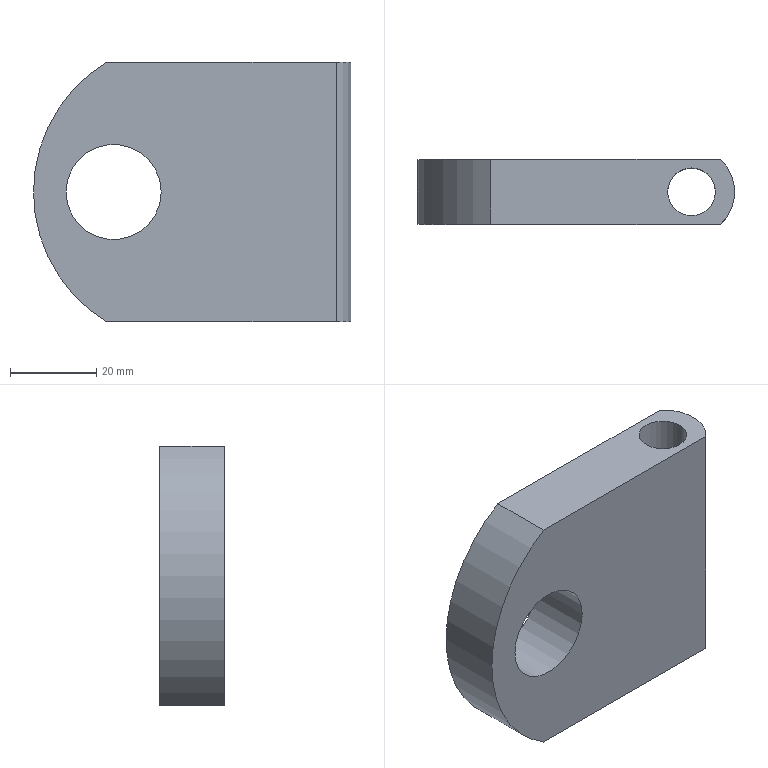Component | NX | MODEL2 | 1 solid | 8 faces | box 73.39 x 15 x 60 mm | volume 49250 mm3 | plane 4 | cylinder 4 | commonest cylinder face diameters 20 x1 11 x1 70.098 x1 22 x1
STEP:
#1=CARTESIAN_POINT('',(0.,0.,0.));
#2=DIRECTION('',(0.,0.,1.));
#3=DIRECTION('',(1.,0.,0.));
#4=AXIS2_PLACEMENT_3D('',#1,#2,#3);
#5=CARTESIAN_POINT('',(-84.997,-51.411,30.));
#6=VERTEX_POINT('',#5);
#7=CARTESIAN_POINT('',(-84.997,-56.911,30.));
#8=DIRECTION('',(0.,0.,1.));
#9=DIRECTION('',(0.,1.,0.));
#10=AXIS2_PLACEMENT_3D('',#7,#8,#9);
#11=CIRCLE('',#10,5.5);
#12=CARTESIAN_POINT('',(-84.997,-56.911,30.));
#13=DIRECTION('',(0.,0.,1.));
#14=DIRECTION('',(1.,0.,0.));
#15=AXIS2_PLACEMENT_3D('',#12,#13,#14);
#16=PLANE('',#15);
#17=CARTESIAN_POINT('',(0.,0.));
#18=DIRECTION('',(0.,1.));
#19=AXIS2_PLACEMENT_2D('',#17,#18);
#20=CIRCLE('',#19,5.5);
#21=(GEOMETRIC_REPRESENTATION_CONTEXT(2)PARAMETRIC_REPRESENTATION_CONTEXT()REPRESENTATION_CONTEXT('',''));
#22=DEFINITIONAL_REPRESENTATION('',(#20),#21);
#23=PCURVE('',#16,#22);
#24=CARTESIAN_POINT('',(-84.997,-56.911,30.));
#25=DIRECTION('',(0.,0.,-1.));
#26=DIRECTION('',(-1.,0.,0.));
#27=AXIS2_PLACEMENT_3D('',#24,#25,#26);
#28=CYLINDRICAL_SURFACE('',#27,5.5);
#29=CARTESIAN_POINT('',(7.854,0.));
#30=DIRECTION('',(-1.,0.));
#31=VECTOR('',#30,1.);
#32=LINE('',#29,#31);
#33=(GEOMETRIC_REPRESENTATION_CONTEXT(2)PARAMETRIC_REPRESENTATION_CONTEXT()REPRESENTATION_CONTEXT('',''));
#34=DEFINITIONAL_REPRESENTATION('',(#32),#33);
#35=PCURVE('',#28,#34);
#36=SURFACE_CURVE('',#11,(#23,#35),.PCURVE_S1.);
#37=EDGE_CURVE('',#6,#6,#36,.T.);
#38=ORIENTED_EDGE('',*,*,#37,.F.);
#39=EDGE_LOOP('',(#38));
#40=FACE_BOUND('',#39,.T.);
#41=CARTESIAN_POINT('',(-78.382,-49.411,30.));
#42=VERTEX_POINT('',#41);
#43=CARTESIAN_POINT('',(-131.456,-49.411,30.));
#44=VERTEX_POINT('',#43);
#45=CARTESIAN_POINT('',(-78.382,-49.411,30.));
#46=DIRECTION('',(-1.,0.,0.));
#47=VECTOR('',#46,1.);
#48=LINE('',#45,#47);
#49=CARTESIAN_POINT('',(6.614,7.5));
#50=DIRECTION('',(-1.,0.));
#51=VECTOR('',#50,1.);
#52=LINE('',#49,#51);
#53=(GEOMETRIC_REPRESENTATION_CONTEXT(2)PARAMETRIC_REPRESENTATION_CONTEXT()REPRESENTATION_CONTEXT('',''));
#54=DEFINITIONAL_REPRESENTATION('',(#52),#53);
#55=PCURVE('',#16,#54);
#56=CARTESIAN_POINT('',(-78.382,-49.411,30.));
#57=DIRECTION('',(-0.,-1.,0.));
#58=DIRECTION('',(1.,-0.,0.));
#59=AXIS2_PLACEMENT_3D('',#56,#57,#58);
#60=PLANE('',#59);
#61=CARTESIAN_POINT('',(0.,0.));
#62=DIRECTION('',(-1.,0.));
#63=VECTOR('',#62,1.);
#64=LINE('',#61,#63);
#65=(GEOMETRIC_REPRESENTATION_CONTEXT(2)PARAMETRIC_REPRESENTATION_CONTEXT()REPRESENTATION_CONTEXT('',''));
#66=DEFINITIONAL_REPRESENTATION('',(#64),#65);
#67=PCURVE('',#60,#66);
#68=SURFACE_CURVE('',#48,(#55,#67),.PCURVE_S1.);
#69=EDGE_CURVE('',#42,#44,#68,.T.);
#70=ORIENTED_EDGE('',*,*,#69,.T.);
#71=CARTESIAN_POINT('',(-131.456,-64.411,30.));
#72=VERTEX_POINT('',#71);
#73=CARTESIAN_POINT('',(-131.456,-19.411,30.));
#74=DIRECTION('',(0.,-1.,0.));
#75=VECTOR('',#74,1.);
#76=LINE('',#73,#75);
#77=CARTESIAN_POINT('',(-46.459,37.5));
#78=DIRECTION('',(0.,-1.));
#79=VECTOR('',#78,1.);
#80=LINE('',#77,#79);
#81=(GEOMETRIC_REPRESENTATION_CONTEXT(2)PARAMETRIC_REPRESENTATION_CONTEXT()REPRESENTATION_CONTEXT('',''));
#82=DEFINITIONAL_REPRESENTATION('',(#80),#81);
#83=PCURVE('',#16,#82);
#84=CARTESIAN_POINT('',(-113.333,-19.411,-0.));
#85=DIRECTION('',(0.,-1.,0.));
#86=DIRECTION('',(1.,0.,0.));
#87=AXIS2_PLACEMENT_3D('',#84,#85,#86);
#88=CYLINDRICAL_SURFACE('',#87,35.049);
#89=CARTESIAN_POINT('',(2.114,0.));
#90=DIRECTION('',(0.,1.));
#91=VECTOR('',#90,1.);
#92=LINE('',#89,#91);
#93=(GEOMETRIC_REPRESENTATION_CONTEXT(2)PARAMETRIC_REPRESENTATION_CONTEXT()REPRESENTATION_CONTEXT('',''));
#94=DEFINITIONAL_REPRESENTATION('',(#92),#93);
#95=PCURVE('',#88,#94);
#96=SURFACE_CURVE('',#76,(#83,#95),.PCURVE_S1.);
#97=EDGE_CURVE('',#44,#72,#96,.T.);
#98=ORIENTED_EDGE('',*,*,#97,.T.);
#99=CARTESIAN_POINT('',(-78.382,-64.411,30.));
#100=VERTEX_POINT('',#99);
#101=CARTESIAN_POINT('',(-148.382,-64.411,30.));
#102=DIRECTION('',(1.,0.,0.));
#103=VECTOR('',#102,1.);
#104=LINE('',#101,#103);
#105=CARTESIAN_POINT('',(-63.386,-7.5));
#106=DIRECTION('',(1.,0.));
#107=VECTOR('',#106,1.);
#108=LINE('',#105,#107);
#109=(GEOMETRIC_REPRESENTATION_CONTEXT(2)PARAMETRIC_REPRESENTATION_CONTEXT()REPRESENTATION_CONTEXT('',''));
#110=DEFINITIONAL_REPRESENTATION('',(#108),#109);
#111=PCURVE('',#16,#110);
#112=CARTESIAN_POINT('',(-148.382,-64.411,30.));
#113=DIRECTION('',(-0.,1.,0.));
#114=DIRECTION('',(-1.,-0.,0.));
#115=AXIS2_PLACEMENT_3D('',#112,#113,#114);
#116=PLANE('',#115);
#117=CARTESIAN_POINT('',(0.,0.));
#118=DIRECTION('',(-1.,0.));
#119=VECTOR('',#118,1.);
#120=LINE('',#117,#119);
#121=(GEOMETRIC_REPRESENTATION_CONTEXT(2)PARAMETRIC_REPRESENTATION_CONTEXT()REPRESENTATION_CONTEXT('',''));
#122=DEFINITIONAL_REPRESENTATION('',(#120),#121);
#123=PCURVE('',#116,#122);
#124=SURFACE_CURVE('',#104,(#111,#123),.PCURVE_S1.);
#125=EDGE_CURVE('',#72,#100,#124,.T.);
#126=ORIENTED_EDGE('',*,*,#125,.T.);
#127=CARTESIAN_POINT('',(-84.997,-56.911,30.));
#128=DIRECTION('',(0.,0.,1.));
#129=DIRECTION('',(0.,1.,0.));
#130=AXIS2_PLACEMENT_3D('',#127,#128,#129);
#131=CIRCLE('',#130,10.);
#132=CARTESIAN_POINT('',(0.,0.));
#133=DIRECTION('',(0.,1.));
#134=AXIS2_PLACEMENT_2D('',#132,#133);
#135=CIRCLE('',#134,10.);
#136=(GEOMETRIC_REPRESENTATION_CONTEXT(2)PARAMETRIC_REPRESENTATION_CONTEXT()REPRESENTATION_CONTEXT('',''));
#137=DEFINITIONAL_REPRESENTATION('',(#135),#136);
#138=PCURVE('',#16,#137);
#139=CARTESIAN_POINT('',(-84.997,-56.911,30.));
#140=DIRECTION('',(0.,0.,-1.));
#141=DIRECTION('',(-1.,0.,0.));
#142=AXIS2_PLACEMENT_3D('',#139,#140,#141);
#143=CYLINDRICAL_SURFACE('',#142,10.);
#144=CARTESIAN_POINT('',(7.854,0.));
#145=DIRECTION('',(-1.,0.));
#146=VECTOR('',#145,1.);
#147=LINE('',#144,#146);
#148=(GEOMETRIC_REPRESENTATION_CONTEXT(2)PARAMETRIC_REPRESENTATION_CONTEXT()REPRESENTATION_CONTEXT('',''));
#149=DEFINITIONAL_REPRESENTATION('',(#147),#148);
#150=PCURVE('',#143,#149);
#151=SURFACE_CURVE('',#131,(#138,#150),.PCURVE_S1.);
#152=EDGE_CURVE('',#100,#42,#151,.T.);
#153=ORIENTED_EDGE('',*,*,#152,.T.);
#154=EDGE_LOOP('',(#70,#98,#126,#153));
#155=FACE_BOUND('',#154,.T.);
#156=ADVANCED_FACE('',(#40,#155),#16,.T.);
#157=CARTESIAN_POINT('',(-84.997,-51.411,-30.));
#158=VERTEX_POINT('',#157);
#159=CARTESIAN_POINT('',(-84.997,-56.911,-30.));
#160=DIRECTION('',(0.,0.,1.));
#161=DIRECTION('',(0.,1.,0.));
#162=AXIS2_PLACEMENT_3D('',#159,#160,#161);
#163=CIRCLE('',#162,5.5);
#164=CARTESIAN_POINT('',(-84.997,-56.911,-30.));
#165=DIRECTION('',(0.,0.,1.));
#166=DIRECTION('',(1.,0.,0.));
#167=AXIS2_PLACEMENT_3D('',#164,#165,#166);
#168=PLANE('',#167);
#169=CARTESIAN_POINT('',(0.,0.));
#170=DIRECTION('',(0.,1.));
#171=AXIS2_PLACEMENT_2D('',#169,#170);
#172=CIRCLE('',#171,5.5);
#173=(GEOMETRIC_REPRESENTATION_CONTEXT(2)PARAMETRIC_REPRESENTATION_CONTEXT()REPRESENTATION_CONTEXT('',''));
#174=DEFINITIONAL_REPRESENTATION('',(#172),#173);
#175=PCURVE('',#168,#174);
#176=CARTESIAN_POINT('',(7.854,60.));
#177=DIRECTION('',(-1.,0.));
#178=VECTOR('',#177,1.);
#179=LINE('',#176,#178);
#180=(GEOMETRIC_REPRESENTATION_CONTEXT(2)PARAMETRIC_REPRESENTATION_CONTEXT()REPRESENTATION_CONTEXT('',''));
#181=DEFINITIONAL_REPRESENTATION('',(#179),#180);
#182=PCURVE('',#28,#181);
#183=SURFACE_CURVE('',#163,(#175,#182),.PCURVE_S1.);
#184=EDGE_CURVE('',#158,#158,#183,.T.);
#185=ORIENTED_EDGE('',*,*,#184,.T.);
#186=EDGE_LOOP('',(#185));
#187=FACE_BOUND('',#186,.T.);
#188=CARTESIAN_POINT('',(-131.456,-49.411,-30.));
#189=VERTEX_POINT('',#188);
#190=CARTESIAN_POINT('',(-131.456,-64.411,-30.));
#191=VERTEX_POINT('',#190);
#192=CARTESIAN_POINT('',(-131.456,-19.411,-30.));
#193=DIRECTION('',(0.,-1.,0.));
#194=VECTOR('',#193,1.);
#195=LINE('',#192,#194);
#196=CARTESIAN_POINT('',(-46.459,37.5));
#197=DIRECTION('',(0.,-1.));
#198=VECTOR('',#197,1.);
#199=LINE('',#196,#198);
#200=(GEOMETRIC_REPRESENTATION_CONTEXT(2)PARAMETRIC_REPRESENTATION_CONTEXT()REPRESENTATION_CONTEXT('',''));
#201=DEFINITIONAL_REPRESENTATION('',(#199),#200);
#202=PCURVE('',#168,#201);
#203=CARTESIAN_POINT('',(4.169,0.));
#204=DIRECTION('',(0.,1.));
#205=VECTOR('',#204,1.);
#206=LINE('',#203,#205);
#207=(GEOMETRIC_REPRESENTATION_CONTEXT(2)PARAMETRIC_REPRESENTATION_CONTEXT()REPRESENTATION_CONTEXT('',''));
#208=DEFINITIONAL_REPRESENTATION('',(#206),#207);
#209=PCURVE('',#88,#208);
#210=SURFACE_CURVE('',#195,(#202,#209),.PCURVE_S1.);
#211=EDGE_CURVE('',#189,#191,#210,.T.);
#212=ORIENTED_EDGE('',*,*,#211,.F.);
#213=CARTESIAN_POINT('',(-78.382,-49.411,-30.));
#214=VERTEX_POINT('',#213);
#215=CARTESIAN_POINT('',(-78.382,-49.411,-30.));
#216=DIRECTION('',(-1.,0.,0.));
#217=VECTOR('',#216,1.);
#218=LINE('',#215,#217);
#219=CARTESIAN_POINT('',(6.614,7.5));
#220=DIRECTION('',(-1.,0.));
#221=VECTOR('',#220,1.);
#222=LINE('',#219,#221);
#223=(GEOMETRIC_REPRESENTATION_CONTEXT(2)PARAMETRIC_REPRESENTATION_CONTEXT()REPRESENTATION_CONTEXT('',''));
#224=DEFINITIONAL_REPRESENTATION('',(#222),#223);
#225=PCURVE('',#168,#224);
#226=CARTESIAN_POINT('',(0.,-60.));
#227=DIRECTION('',(-1.,0.));
#228=VECTOR('',#227,1.);
#229=LINE('',#226,#228);
#230=(GEOMETRIC_REPRESENTATION_CONTEXT(2)PARAMETRIC_REPRESENTATION_CONTEXT()REPRESENTATION_CONTEXT('',''));
#231=DEFINITIONAL_REPRESENTATION('',(#229),#230);
#232=PCURVE('',#60,#231);
#233=SURFACE_CURVE('',#218,(#225,#232),.PCURVE_S1.);
#234=EDGE_CURVE('',#214,#189,#233,.T.);
#235=ORIENTED_EDGE('',*,*,#234,.F.);
#236=CARTESIAN_POINT('',(-78.382,-64.411,-30.));
#237=VERTEX_POINT('',#236);
#238=CARTESIAN_POINT('',(-84.997,-56.911,-30.));
#239=DIRECTION('',(0.,0.,1.));
#240=DIRECTION('',(0.,1.,0.));
#241=AXIS2_PLACEMENT_3D('',#238,#239,#240);
#242=CIRCLE('',#241,10.);
#243=CARTESIAN_POINT('',(0.,0.));
#244=DIRECTION('',(0.,1.));
#245=AXIS2_PLACEMENT_2D('',#243,#244);
#246=CIRCLE('',#245,10.);
#247=(GEOMETRIC_REPRESENTATION_CONTEXT(2)PARAMETRIC_REPRESENTATION_CONTEXT()REPRESENTATION_CONTEXT('',''));
#248=DEFINITIONAL_REPRESENTATION('',(#246),#247);
#249=PCURVE('',#168,#248);
#250=CARTESIAN_POINT('',(7.854,60.));
#251=DIRECTION('',(-1.,0.));
#252=VECTOR('',#251,1.);
#253=LINE('',#250,#252);
#254=(GEOMETRIC_REPRESENTATION_CONTEXT(2)PARAMETRIC_REPRESENTATION_CONTEXT()REPRESENTATION_CONTEXT('',''));
#255=DEFINITIONAL_REPRESENTATION('',(#253),#254);
#256=PCURVE('',#143,#255);
#257=SURFACE_CURVE('',#242,(#249,#256),.PCURVE_S1.);
#258=EDGE_CURVE('',#237,#214,#257,.T.);
#259=ORIENTED_EDGE('',*,*,#258,.F.);
#260=CARTESIAN_POINT('',(-148.382,-64.411,-30.));
#261=DIRECTION('',(1.,0.,0.));
#262=VECTOR('',#261,1.);
#263=LINE('',#260,#262);
#264=CARTESIAN_POINT('',(-63.386,-7.5));
#265=DIRECTION('',(1.,0.));
#266=VECTOR('',#265,1.);
#267=LINE('',#264,#266);
#268=(GEOMETRIC_REPRESENTATION_CONTEXT(2)PARAMETRIC_REPRESENTATION_CONTEXT()REPRESENTATION_CONTEXT('',''));
#269=DEFINITIONAL_REPRESENTATION('',(#267),#268);
#270=PCURVE('',#168,#269);
#271=CARTESIAN_POINT('',(0.,-60.));
#272=DIRECTION('',(-1.,0.));
#273=VECTOR('',#272,1.);
#274=LINE('',#271,#273);
#275=(GEOMETRIC_REPRESENTATION_CONTEXT(2)PARAMETRIC_REPRESENTATION_CONTEXT()REPRESENTATION_CONTEXT('',''));
#276=DEFINITIONAL_REPRESENTATION('',(#274),#275);
#277=PCURVE('',#116,#276);
#278=SURFACE_CURVE('',#263,(#270,#277),.PCURVE_S1.);
#279=EDGE_CURVE('',#191,#237,#278,.T.);
#280=ORIENTED_EDGE('',*,*,#279,.F.);
#281=EDGE_LOOP('',(#212,#235,#259,#280));
#282=FACE_BOUND('',#281,.T.);
#283=ADVANCED_FACE('',(#187,#282),#168,.F.);
#284=CARTESIAN_POINT('',(-118.847,-49.411,-0.));
#285=VERTEX_POINT('',#284);
#286=CARTESIAN_POINT('',(-129.847,-49.411,-0.));
#287=DIRECTION('',(0.,1.,0.));
#288=DIRECTION('',(1.,-0.,0.));
#289=AXIS2_PLACEMENT_3D('',#286,#287,#288);
#290=CIRCLE('',#289,11.);
#291=CARTESIAN_POINT('',(-40.464,-30.));
#292=CARTESIAN_POINT('',(-40.464,-49.053));
#293=CARTESIAN_POINT('',(-56.964,-39.526));
#294=CARTESIAN_POINT('',(-73.464,-30.));
#295=CARTESIAN_POINT('',(-56.964,-20.474));
#296=CARTESIAN_POINT('',(-40.464,-10.947));
#297=CARTESIAN_POINT('',(-40.464,-30.));
#298=(BOUNDED_CURVE()B_SPLINE_CURVE(2,(#291,#292,#293,#294,#295,#296,#297),.UNSPECIFIED.,.T.,.F.)B_SPLINE_CURVE_WITH_KNOTS((1,2,2,2,2,1),(-2.094,0.,2.094,4.189,6.283,8.378),.UNSPECIFIED.)CURVE()GEOMETRIC_REPRESENTATION_ITEM()RATIONAL_B_SPLINE_CURVE((1.,0.5,1.,0.5,1.,0.5,1.))REPRESENTATION_ITEM(''));
#299=(GEOMETRIC_REPRESENTATION_CONTEXT(2)PARAMETRIC_REPRESENTATION_CONTEXT()REPRESENTATION_CONTEXT('',''));
#300=DEFINITIONAL_REPRESENTATION('',(#298),#299);
#301=PCURVE('',#60,#300);
#302=CARTESIAN_POINT('',(-129.847,-19.411,-0.));
#303=DIRECTION('',(0.,-1.,0.));
#304=DIRECTION('',(1.,0.,0.));
#305=AXIS2_PLACEMENT_3D('',#302,#303,#304);
#306=CYLINDRICAL_SURFACE('',#305,11.);
#307=CARTESIAN_POINT('',(6.283,30.));
#308=DIRECTION('',(-1.,0.));
#309=VECTOR('',#308,1.);
#310=LINE('',#307,#309);
#311=(GEOMETRIC_REPRESENTATION_CONTEXT(2)PARAMETRIC_REPRESENTATION_CONTEXT()REPRESENTATION_CONTEXT('',''));
#312=DEFINITIONAL_REPRESENTATION('',(#310),#311);
#313=PCURVE('',#306,#312);
#314=SURFACE_CURVE('',#290,(#301,#313),.PCURVE_S1.);
#315=EDGE_CURVE('',#285,#285,#314,.T.);
#316=ORIENTED_EDGE('',*,*,#315,.F.);
#317=EDGE_LOOP('',(#316));
#318=FACE_BOUND('',#317,.T.);
#319=CARTESIAN_POINT('',(-113.333,-49.411,-0.));
#320=DIRECTION('',(-0.,-1.,0.));
#321=DIRECTION('',(1.,-0.,0.));
#322=AXIS2_PLACEMENT_3D('',#319,#320,#321);
#323=CIRCLE('',#322,35.049);
#324=CARTESIAN_POINT('',(-34.951,-30.));
#325=DIRECTION('',(1.,0.));
#326=AXIS2_PLACEMENT_2D('',#324,#325);
#327=CIRCLE('',#326,35.049);
#328=(GEOMETRIC_REPRESENTATION_CONTEXT(2)PARAMETRIC_REPRESENTATION_CONTEXT()REPRESENTATION_CONTEXT('',''));
#329=DEFINITIONAL_REPRESENTATION('',(#327),#328);
#330=PCURVE('',#60,#329);
#331=CARTESIAN_POINT('',(-0.,30.));
#332=DIRECTION('',(1.,0.));
#333=VECTOR('',#332,1.);
#334=LINE('',#331,#333);
#335=(GEOMETRIC_REPRESENTATION_CONTEXT(2)PARAMETRIC_REPRESENTATION_CONTEXT()REPRESENTATION_CONTEXT('',''));
#336=DEFINITIONAL_REPRESENTATION('',(#334),#335);
#337=PCURVE('',#88,#336);
#338=SURFACE_CURVE('',#323,(#330,#337),.PCURVE_S1.);
#339=EDGE_CURVE('',#44,#189,#338,.T.);
#340=ORIENTED_EDGE('',*,*,#339,.F.);
#341=ORIENTED_EDGE('',*,*,#69,.F.);
#342=CARTESIAN_POINT('',(-78.382,-49.411,30.));
#343=DIRECTION('',(0.,0.,-1.));
#344=VECTOR('',#343,1.);
#345=LINE('',#342,#344);
#346=CARTESIAN_POINT('',(0.,0.));
#347=DIRECTION('',(0.,-1.));
#348=VECTOR('',#347,1.);
#349=LINE('',#346,#348);
#350=(GEOMETRIC_REPRESENTATION_CONTEXT(2)PARAMETRIC_REPRESENTATION_CONTEXT()REPRESENTATION_CONTEXT('',''));
#351=DEFINITIONAL_REPRESENTATION('',(#349),#350);
#352=PCURVE('',#60,#351);
#353=CARTESIAN_POINT('',(2.294,0.));
#354=DIRECTION('',(0.,1.));
#355=VECTOR('',#354,1.);
#356=LINE('',#353,#355);
#357=(GEOMETRIC_REPRESENTATION_CONTEXT(2)PARAMETRIC_REPRESENTATION_CONTEXT()REPRESENTATION_CONTEXT('',''));
#358=DEFINITIONAL_REPRESENTATION('',(#356),#357);
#359=PCURVE('',#143,#358);
#360=SURFACE_CURVE('',#345,(#352,#359),.PCURVE_S1.);
#361=EDGE_CURVE('',#42,#214,#360,.T.);
#362=ORIENTED_EDGE('',*,*,#361,.T.);
#363=ORIENTED_EDGE('',*,*,#234,.T.);
#364=EDGE_LOOP('',(#340,#341,#362,#363));
#365=FACE_BOUND('',#364,.T.);
#366=ADVANCED_FACE('',(#318,#365),#60,.F.);
#367=CARTESIAN_POINT('',(-140.847,-64.411,-0.));
#368=VERTEX_POINT('',#367);
#369=CARTESIAN_POINT('',(-118.847,-64.411,-0.));
#370=VERTEX_POINT('',#369);
#371=CARTESIAN_POINT('',(-129.847,-64.411,-0.));
#372=DIRECTION('',(0.,-1.,0.));
#373=DIRECTION('',(-1.,-0.,0.));
#374=AXIS2_PLACEMENT_3D('',#371,#372,#373);
#375=CIRCLE('',#374,11.);
#376=CARTESIAN_POINT('',(-7.536,-30.));
#377=CARTESIAN_POINT('',(-7.536,-49.053));
#378=CARTESIAN_POINT('',(-24.036,-39.526));
#379=CARTESIAN_POINT('',(-40.536,-30.));
#380=CARTESIAN_POINT('',(-24.036,-20.474));
#381=CARTESIAN_POINT('',(-7.536,-10.947));
#382=CARTESIAN_POINT('',(-7.536,-30.));
#383=(BOUNDED_CURVE()B_SPLINE_CURVE(2,(#376,#377,#378,#379,#380,#381,#382),.UNSPECIFIED.,.T.,.F.)B_SPLINE_CURVE_WITH_KNOTS((1,2,2,2,2,1),(-2.094,0.,2.094,4.189,6.283,8.378),.UNSPECIFIED.)CURVE()GEOMETRIC_REPRESENTATION_ITEM()RATIONAL_B_SPLINE_CURVE((1.,0.5,1.,0.5,1.,0.5,1.))REPRESENTATION_ITEM(''));
#384=(GEOMETRIC_REPRESENTATION_CONTEXT(2)PARAMETRIC_REPRESENTATION_CONTEXT()REPRESENTATION_CONTEXT('',''));
#385=DEFINITIONAL_REPRESENTATION('',(#383),#384);
#386=PCURVE('',#116,#385);
#387=CARTESIAN_POINT('',(3.142,45.));
#388=DIRECTION('',(1.,0.));
#389=VECTOR('',#388,1.);
#390=LINE('',#387,#389);
#391=(GEOMETRIC_REPRESENTATION_CONTEXT(2)PARAMETRIC_REPRESENTATION_CONTEXT()REPRESENTATION_CONTEXT('',''));
#392=DEFINITIONAL_REPRESENTATION('',(#390),#391);
#393=PCURVE('',#306,#392);
#394=SURFACE_CURVE('',#375,(#386,#393),.PCURVE_S1.);
#395=EDGE_CURVE('',#368,#370,#394,.T.);
#396=ORIENTED_EDGE('',*,*,#395,.F.);
#397=CARTESIAN_POINT('',(-129.847,-64.411,-0.));
#398=DIRECTION('',(0.,-1.,0.));
#399=DIRECTION('',(-1.,-0.,0.));
#400=AXIS2_PLACEMENT_3D('',#397,#398,#399);
#401=CIRCLE('',#400,11.);
#402=CARTESIAN_POINT('',(-7.536,-30.));
#403=CARTESIAN_POINT('',(-7.536,-49.053));
#404=CARTESIAN_POINT('',(-24.036,-39.526));
#405=CARTESIAN_POINT('',(-40.536,-30.));
#406=CARTESIAN_POINT('',(-24.036,-20.474));
#407=CARTESIAN_POINT('',(-7.536,-10.947));
#408=CARTESIAN_POINT('',(-7.536,-30.));
#409=(BOUNDED_CURVE()B_SPLINE_CURVE(2,(#402,#403,#404,#405,#406,#407,#408),.UNSPECIFIED.,.T.,.F.)B_SPLINE_CURVE_WITH_KNOTS((1,2,2,2,2,1),(-2.094,0.,2.094,4.189,6.283,8.378),.UNSPECIFIED.)CURVE()GEOMETRIC_REPRESENTATION_ITEM()RATIONAL_B_SPLINE_CURVE((1.,0.5,1.,0.5,1.,0.5,1.))REPRESENTATION_ITEM(''));
#410=(GEOMETRIC_REPRESENTATION_CONTEXT(2)PARAMETRIC_REPRESENTATION_CONTEXT()REPRESENTATION_CONTEXT('',''));
#411=DEFINITIONAL_REPRESENTATION('',(#409),#410);
#412=PCURVE('',#116,#411);
#413=CARTESIAN_POINT('',(-3.142,45.));
#414=DIRECTION('',(1.,0.));
#415=VECTOR('',#414,1.);
#416=LINE('',#413,#415);
#417=(GEOMETRIC_REPRESENTATION_CONTEXT(2)PARAMETRIC_REPRESENTATION_CONTEXT()REPRESENTATION_CONTEXT('',''));
#418=DEFINITIONAL_REPRESENTATION('',(#416),#417);
#419=PCURVE('',#306,#418);
#420=SURFACE_CURVE('',#401,(#412,#419),.PCURVE_S1.);
#421=EDGE_CURVE('',#370,#368,#420,.T.);
#422=ORIENTED_EDGE('',*,*,#421,.F.);
#423=EDGE_LOOP('',(#396,#422));
#424=FACE_BOUND('',#423,.T.);
#425=ORIENTED_EDGE('',*,*,#125,.F.);
#426=CARTESIAN_POINT('',(-113.333,-64.411,-0.));
#427=DIRECTION('',(-0.,1.,0.));
#428=DIRECTION('',(-1.,-0.,0.));
#429=AXIS2_PLACEMENT_3D('',#426,#427,#428);
#430=CIRCLE('',#429,35.049);
#431=CARTESIAN_POINT('',(-35.049,-30.));
#432=DIRECTION('',(1.,0.));
#433=AXIS2_PLACEMENT_2D('',#431,#432);
#434=CIRCLE('',#433,35.049);
#435=(GEOMETRIC_REPRESENTATION_CONTEXT(2)PARAMETRIC_REPRESENTATION_CONTEXT()REPRESENTATION_CONTEXT('',''));
#436=DEFINITIONAL_REPRESENTATION('',(#434),#435);
#437=PCURVE('',#116,#436);
#438=CARTESIAN_POINT('',(9.425,45.));
#439=DIRECTION('',(-1.,0.));
#440=VECTOR('',#439,1.);
#441=LINE('',#438,#440);
#442=(GEOMETRIC_REPRESENTATION_CONTEXT(2)PARAMETRIC_REPRESENTATION_CONTEXT()REPRESENTATION_CONTEXT('',''));
#443=DEFINITIONAL_REPRESENTATION('',(#441),#442);
#444=PCURVE('',#88,#443);
#445=SURFACE_CURVE('',#430,(#437,#444),.PCURVE_S1.);
#446=EDGE_CURVE('',#191,#72,#445,.T.);
#447=ORIENTED_EDGE('',*,*,#446,.F.);
#448=ORIENTED_EDGE('',*,*,#279,.T.);
#449=CARTESIAN_POINT('',(-78.382,-64.411,30.));
#450=DIRECTION('',(0.,0.,-1.));
#451=VECTOR('',#450,1.);
#452=LINE('',#449,#451);
#453=CARTESIAN_POINT('',(-70.,0.));
#454=DIRECTION('',(0.,-1.));
#455=VECTOR('',#454,1.);
#456=LINE('',#453,#455);
#457=(GEOMETRIC_REPRESENTATION_CONTEXT(2)PARAMETRIC_REPRESENTATION_CONTEXT()REPRESENTATION_CONTEXT('',''));
#458=DEFINITIONAL_REPRESENTATION('',(#456),#457);
#459=PCURVE('',#116,#458);
#460=CARTESIAN_POINT('',(3.99,0.));
#461=DIRECTION('',(0.,1.));
#462=VECTOR('',#461,1.);
#463=LINE('',#460,#462);
#464=(GEOMETRIC_REPRESENTATION_CONTEXT(2)PARAMETRIC_REPRESENTATION_CONTEXT()REPRESENTATION_CONTEXT('',''));
#465=DEFINITIONAL_REPRESENTATION('',(#463),#464);
#466=PCURVE('',#143,#465);
#467=SURFACE_CURVE('',#452,(#459,#466),.PCURVE_S1.);
#468=EDGE_CURVE('',#100,#237,#467,.T.);
#469=ORIENTED_EDGE('',*,*,#468,.F.);
#470=EDGE_LOOP('',(#425,#447,#448,#469));
#471=FACE_BOUND('',#470,.T.);
#472=ADVANCED_FACE('',(#424,#471),#116,.F.);
#473=ORIENTED_EDGE('',*,*,#258,.T.);
#474=ORIENTED_EDGE('',*,*,#361,.F.);
#475=ORIENTED_EDGE('',*,*,#152,.F.);
#476=ORIENTED_EDGE('',*,*,#468,.T.);
#477=EDGE_LOOP('',(#473,#474,#475,#476));
#478=FACE_BOUND('',#477,.T.);
#479=ADVANCED_FACE('',(#478),#143,.T.);
#480=ORIENTED_EDGE('',*,*,#37,.F.);
#481=CARTESIAN_POINT('',(-84.997,-51.411,30.));
#482=CARTESIAN_POINT('',(-84.997,-51.411,-30.));
#483=B_SPLINE_CURVE_WITH_KNOTS('',1,(#481,#482),.UNSPECIFIED.,.F.,.F.,(2,2),(0.,60.),.PIECEWISE_BEZIER_KNOTS.);
#484=CARTESIAN_POINT('',(7.854,0.));
#485=DIRECTION('',(0.,1.));
#486=VECTOR('',#485,1.);
#487=LINE('',#484,#486);
#488=(GEOMETRIC_REPRESENTATION_CONTEXT(2)PARAMETRIC_REPRESENTATION_CONTEXT()REPRESENTATION_CONTEXT('',''));
#489=DEFINITIONAL_REPRESENTATION('',(#487),#488);
#490=PCURVE('',#28,#489);
#491=CARTESIAN_POINT('',(1.571,0.));
#492=DIRECTION('',(0.,1.));
#493=VECTOR('',#492,1.);
#494=LINE('',#491,#493);
#495=(GEOMETRIC_REPRESENTATION_CONTEXT(2)PARAMETRIC_REPRESENTATION_CONTEXT()REPRESENTATION_CONTEXT('',''));
#496=DEFINITIONAL_REPRESENTATION('',(#494),#495);
#497=PCURVE('',#28,#496);
#498=SEAM_CURVE('',#483,(#490,#497),.PCURVE_S1.);
#499=EDGE_CURVE('',#6,#158,#498,.T.);
#500=ORIENTED_EDGE('',*,*,#499,.T.);
#501=ORIENTED_EDGE('',*,*,#184,.T.);
#502=ORIENTED_EDGE('',*,*,#499,.F.);
#503=EDGE_LOOP('',(#480,#500,#501,#502));
#504=FACE_BOUND('',#503,.F.);
#505=ADVANCED_FACE('',(#504),#28,.F.);
#506=ORIENTED_EDGE('',*,*,#339,.T.);
#507=ORIENTED_EDGE('',*,*,#211,.T.);
#508=ORIENTED_EDGE('',*,*,#446,.T.);
#509=ORIENTED_EDGE('',*,*,#97,.F.);
#510=EDGE_LOOP('',(#506,#507,#508,#509));
#511=FACE_BOUND('',#510,.T.);
#512=ADVANCED_FACE('',(#511),#88,.T.);
#513=ORIENTED_EDGE('',*,*,#421,.F.);
#514=CARTESIAN_POINT('',(-118.847,-49.411,-0.));
#515=CARTESIAN_POINT('',(-118.847,-64.411,-0.));
#516=B_SPLINE_CURVE_WITH_KNOTS('',1,(#514,#515),.UNSPECIFIED.,.F.,.F.,(2,2),(30.,45.),.PIECEWISE_BEZIER_KNOTS.);
#517=CARTESIAN_POINT('',(0.,0.));
#518=DIRECTION('',(0.,1.));
#519=VECTOR('',#518,1.);
#520=LINE('',#517,#519);
#521=(GEOMETRIC_REPRESENTATION_CONTEXT(2)PARAMETRIC_REPRESENTATION_CONTEXT()REPRESENTATION_CONTEXT('',''));
#522=DEFINITIONAL_REPRESENTATION('',(#520),#521);
#523=PCURVE('',#306,#522);
#524=CARTESIAN_POINT('',(6.283,0.));
#525=DIRECTION('',(0.,1.));
#526=VECTOR('',#525,1.);
#527=LINE('',#524,#526);
#528=(GEOMETRIC_REPRESENTATION_CONTEXT(2)PARAMETRIC_REPRESENTATION_CONTEXT()REPRESENTATION_CONTEXT('',''));
#529=DEFINITIONAL_REPRESENTATION('',(#527),#528);
#530=PCURVE('',#306,#529);
#531=SEAM_CURVE('',#516,(#523,#530),.PCURVE_S1.);
#532=EDGE_CURVE('',#285,#370,#531,.T.);
#533=ORIENTED_EDGE('',*,*,#532,.F.);
#534=ORIENTED_EDGE('',*,*,#315,.F.);
#535=ORIENTED_EDGE('',*,*,#532,.T.);
#536=ORIENTED_EDGE('',*,*,#395,.F.);
#537=EDGE_LOOP('',(#513,#533,#534,#535,#536));
#538=FACE_BOUND('',#537,.F.);
#539=ADVANCED_FACE('',(#538),#306,.F.);
#540=CLOSED_SHELL('',(#156,#283,#366,#472,#479,#505,#512,#539));
#541=MANIFOLD_SOLID_BREP('',#540);
#542=(LENGTH_UNIT()NAMED_UNIT(*)SI_UNIT(.MILLI.,.METRE.));
#543=UNCERTAINTY_MEASURE_WITH_UNIT(LENGTH_MEASURE(0.000002),#542,'','');
#544=(NAMED_UNIT(*)PLANE_ANGLE_UNIT()SI_UNIT($,.RADIAN.));
#545=(NAMED_UNIT(*)SI_UNIT($,.STERADIAN.)SOLID_ANGLE_UNIT());
#546=(GEOMETRIC_REPRESENTATION_CONTEXT(3)GLOBAL_UNCERTAINTY_ASSIGNED_CONTEXT((#543))GLOBAL_UNIT_ASSIGNED_CONTEXT((#542,#544,#545))REPRESENTATION_CONTEXT('',''));
#547=ADVANCED_BREP_SHAPE_REPRESENTATION('',(#4,#541),#546);